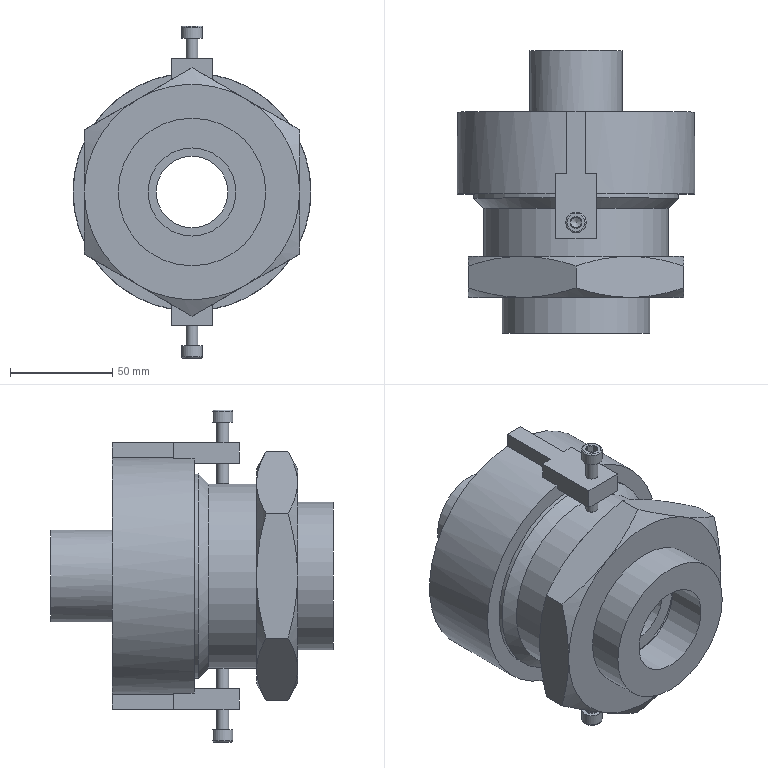Assembly | NX | mm | 8 component files | 8 solids | 138 faces | box 116 x 138 x 162 mm | volume 735733 mm3 | plane 75 | cone 29 | cylinder 26 | sphere 4 | torus 4 | commonest cylinder face diameters 5.795 x4 80 x4 35 x2 10 x2 116 x2 100 x2 55 x2 45 x1
Bill of materials:
unnamed part 1 | 1 |  | Short cylindrical ring band with two rectangular lugs on opposite sides of the outside diameter. Each lug has one small through hole.
unnamed part 2 | 1 |  | Plain thick-walled annular ring with a through bore. It looks like a spacer or washer.
unnamed part 3 | 1 |  | Thin-walled, narrow annular ring with a large bore relative to its outside diameter.
unnamed part 4 | 1 |  | Turned body with a central hexagonal flange. It has a stepped cylindrical section on one side, a smaller cylindrical spigot on the other side, and a through bore along the axis.
unnamed part 5 | 1 |  | Spherical body cut flat on one side, with a coaxial cylindrical tubular shank on the opposite side. A through bore runs along the common axis.
GB-T70.1-2000,M6x30 | 2 |  | Hexagon Socket Head Cap Screw, GB-T 70.1-2000,M6x30
unnamed part 6 | 1 |  | Thin-walled cylindrical sleeve or ring. The inside appears to be stepped or tapered.
Mates:
1. concentric | Shim 1 edge | Movable_Pad 1 edge
2. concentric | Fixed_Pad 1 edge | Shim 1 edge
3. touch align | Ball_Joint 1 face | Shim 1 face
4. concentric | Movable_Pad 1 edge | Cap_Nut 1 edge
5. concentric | Fixed_Pad 1 edge | Hinge_Body 1 edge
6. touch align | Screw_M6x30 2 face | Cap_Nut 1 face
7. touch align | Screw_M6x30 2 face | Hinge_Body 1 face
8. bond | Cap_Nut 1 component | assembly component
9. bond | Screw_M6x30 2 component | assembly component
10. bond | Screw_M6x30 1 component | assembly component
11. circular | assembly datumaxis | assembly cartesiancoordinatesystem | assembly cartesiancoordinatesystem